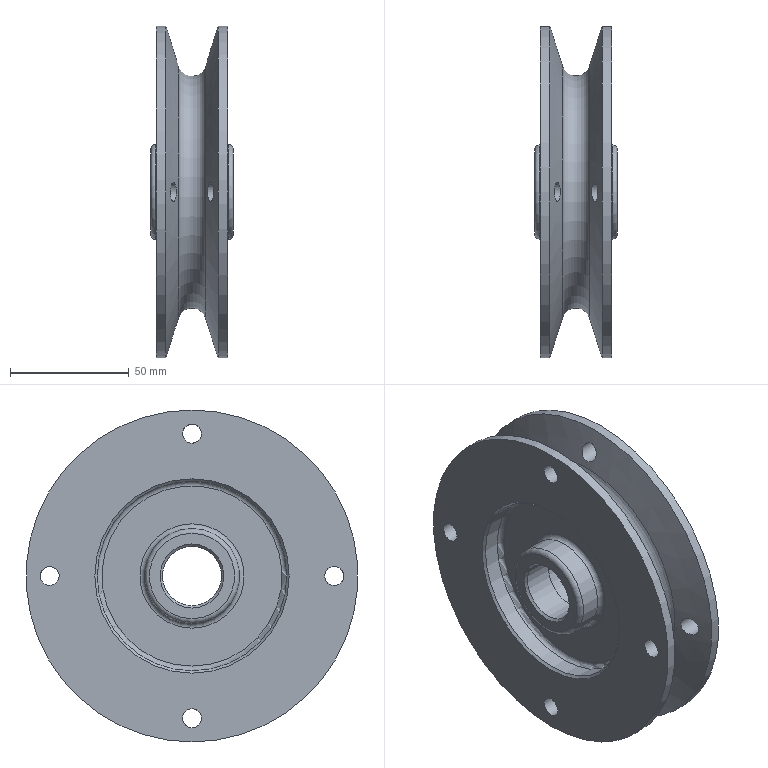Component | NX | 5_PULLEY | 1 solid | 38 faces | volume 249688 mm3 | cylinder 17 | plane 8 | torus 7 | cone 6 | commonest cylinder face diameters 8 x8 25 x2 40 x2 80 x2 140 x2 29 x1